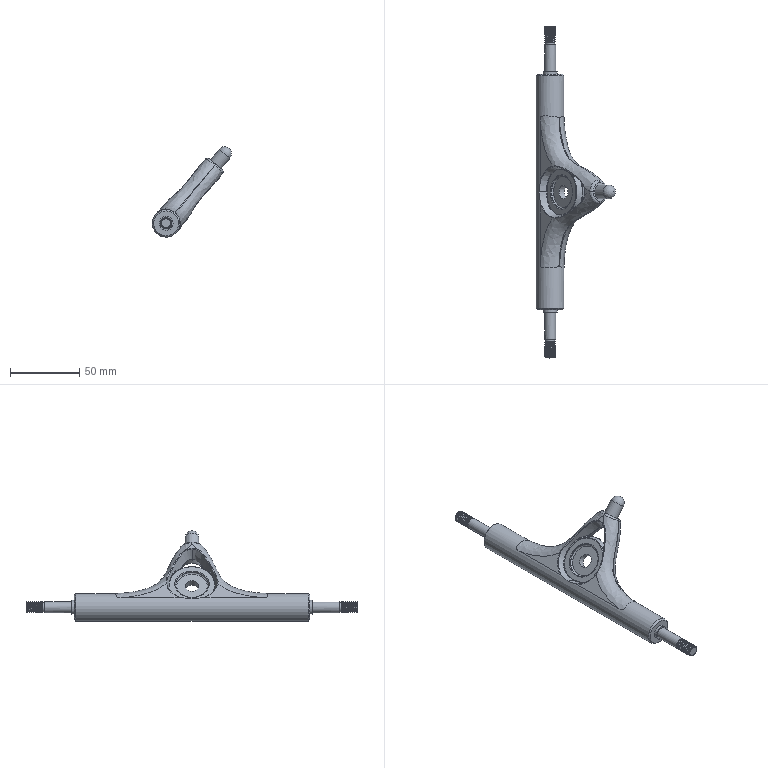Component | NX | HANGER_2 | 1 solid | 115 faces | volume 75612 mm3 | spline 48 | cylinder 30 | plane 21 | torus 7 | cone 6 | other 2 | sphere 1 | commonest cylinder face diameters 6.53 x18 10 x4 8 x4 24 x2 20 x1 4 x1